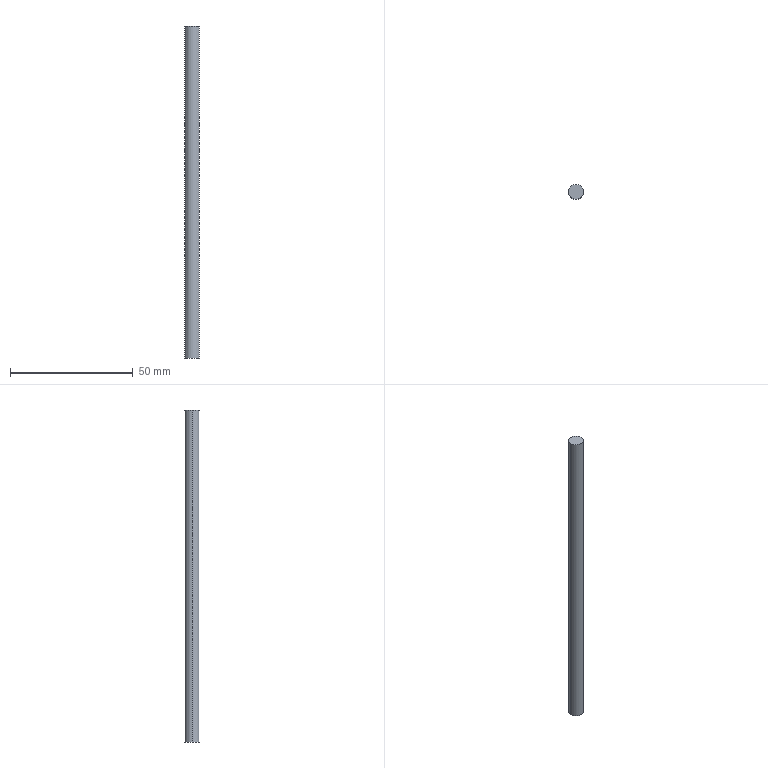Component | SolidWorks | Assembly5.1-1_TailstockAxisBar.1-1 | 1 solid | 4 faces | box 6 x 6 x 135 mm | volume 3817 mm3 | cylinder 2 | plane 2 | commonest cylinder face diameters 6 x2
build123d program:
from build123d import *

# Parameters (mm, degrees)
SKETCH1_R           = 3
BOSS_EXTRUDE1_DEPTH = 67.5


with BuildPart() as part:
    # Sketch1 → Boss-Extrude1 (new, symmetric)
    with BuildSketch(Plane.XY):
        Circle(SKETCH1_R)
    extrude(amount=BOSS_EXTRUDE1_DEPTH, both=True)


solid = part.part

# Placed as in the assembly
solid = solid.moved(Location((70, 164, 0), (0, 0, 0)))
STEP:
#1=COLOUR_RGB('',0.7922,0.8196,0.9333);
#2=FILL_AREA_STYLE_COLOUR('',#1);
#3=FILL_AREA_STYLE('',(#2));
#4=SURFACE_STYLE_FILL_AREA(#3);
#5=SURFACE_SIDE_STYLE('',(#4));
#6=SURFACE_STYLE_USAGE(.BOTH.,#5);
#7=PRESENTATION_STYLE_ASSIGNMENT((#6));
#8=CARTESIAN_POINT('',(2.874,6.457,2.657));
#9=VERTEX_POINT('',#8);
#10=CARTESIAN_POINT('',(2.638,6.457,2.657));
#11=VERTEX_POINT('',#10);
#12=CARTESIAN_POINT('',(2.756,6.457,2.657));
#13=DIRECTION('',(0.,0.,1.));
#14=DIRECTION('',(1.,0.,0.));
#15=AXIS2_PLACEMENT_3D('',#12,#13,#14);
#16=CIRCLE('',#15,0.1181);
#17=EDGE_CURVE('',#9,#11,#16,.T.);
#18=ORIENTED_EDGE('',*,*,#17,.F.);
#19=CARTESIAN_POINT('',(2.874,6.457,-2.657));
#20=VERTEX_POINT('',#19);
#21=CARTESIAN_POINT('',(2.874,6.457,2.657));
#22=DIRECTION('',(0.,0.,-1.));
#23=VECTOR('',#22,39.37);
#24=LINE('',#21,#23);
#25=EDGE_CURVE('',#9,#20,#24,.T.);
#26=ORIENTED_EDGE('',*,*,#25,.T.);
#27=CARTESIAN_POINT('',(2.638,6.457,-2.657));
#28=VERTEX_POINT('',#27);
#29=CARTESIAN_POINT('',(2.756,6.457,-2.657));
#30=DIRECTION('',(0.,0.,1.));
#31=DIRECTION('',(1.,0.,0.));
#32=AXIS2_PLACEMENT_3D('',#29,#30,#31);
#33=CIRCLE('',#32,0.1181);
#34=EDGE_CURVE('',#20,#28,#33,.T.);
#35=ORIENTED_EDGE('',*,*,#34,.T.);
#36=CARTESIAN_POINT('',(2.638,6.457,2.657));
#37=DIRECTION('',(0.,0.,-1.));
#38=VECTOR('',#37,39.37);
#39=LINE('',#36,#38);
#40=EDGE_CURVE('',#11,#28,#39,.T.);
#41=ORIENTED_EDGE('',*,*,#40,.F.);
#42=EDGE_LOOP('',(#18,#26,#35,#41));
#43=FACE_OUTER_BOUND('',#42,.T.);
#44=CARTESIAN_POINT('',(2.756,6.457,2.657));
#45=DIRECTION('',(0.,0.,-1.));
#46=DIRECTION('',(-1.,0.,0.));
#47=AXIS2_PLACEMENT_3D('',#44,#45,#46);
#48=CYLINDRICAL_SURFACE('',#47,0.1181);
#49=ADVANCED_FACE('',(#43),#48,.T.);
#50=ORIENTED_EDGE('',*,*,#25,.F.);
#51=CARTESIAN_POINT('',(2.756,6.457,2.657));
#52=DIRECTION('',(0.,0.,1.));
#53=DIRECTION('',(1.,0.,0.));
#54=AXIS2_PLACEMENT_3D('',#51,#52,#53);
#55=CIRCLE('',#54,0.1181);
#56=EDGE_CURVE('',#11,#9,#55,.T.);
#57=ORIENTED_EDGE('',*,*,#56,.F.);
#58=ORIENTED_EDGE('',*,*,#40,.T.);
#59=CARTESIAN_POINT('',(2.756,6.457,-2.657));
#60=DIRECTION('',(0.,0.,1.));
#61=DIRECTION('',(1.,0.,0.));
#62=AXIS2_PLACEMENT_3D('',#59,#60,#61);
#63=CIRCLE('',#62,0.1181);
#64=EDGE_CURVE('',#28,#20,#63,.T.);
#65=ORIENTED_EDGE('',*,*,#64,.T.);
#66=EDGE_LOOP('',(#50,#57,#58,#65));
#67=FACE_OUTER_BOUND('',#66,.T.);
#68=CARTESIAN_POINT('',(2.756,6.457,2.657));
#69=DIRECTION('',(0.,0.,-1.));
#70=DIRECTION('',(-1.,0.,0.));
#71=AXIS2_PLACEMENT_3D('',#68,#69,#70);
#72=CYLINDRICAL_SURFACE('',#71,0.1181);
#73=ADVANCED_FACE('',(#67),#72,.T.);
#74=ORIENTED_EDGE('',*,*,#56,.T.);
#75=ORIENTED_EDGE('',*,*,#17,.T.);
#76=EDGE_LOOP('',(#74,#75));
#77=FACE_OUTER_BOUND('',#76,.T.);
#78=CARTESIAN_POINT('',(2.756,6.457,2.657));
#79=DIRECTION('',(0.,0.,1.));
#80=DIRECTION('',(1.,0.,0.));
#81=AXIS2_PLACEMENT_3D('',#78,#79,#80);
#82=PLANE('',#81);
#83=ADVANCED_FACE('',(#77),#82,.T.);
#84=ORIENTED_EDGE('',*,*,#64,.F.);
#85=ORIENTED_EDGE('',*,*,#34,.F.);
#86=EDGE_LOOP('',(#84,#85));
#87=FACE_OUTER_BOUND('',#86,.T.);
#88=CARTESIAN_POINT('',(2.756,6.457,-2.657));
#89=DIRECTION('',(0.,0.,1.));
#90=DIRECTION('',(1.,0.,0.));
#91=AXIS2_PLACEMENT_3D('',#88,#89,#90);
#92=PLANE('',#91);
#93=ADVANCED_FACE('',(#87),#92,.F.);
#94=CLOSED_SHELL('',(#49,#73,#83,#93));
#95=MANIFOLD_SOLID_BREP('',#94);
#96=STYLED_ITEM('',(#7),#95);
#97=PRESENTATION_LAYER_ASSIGNMENT('','',(#96));
#98=(LENGTH_UNIT()NAMED_UNIT(*)SI_UNIT($,.METRE.));
#99=LENGTH_MEASURE_WITH_UNIT(LENGTH_MEASURE(0.0254),#98);
#100=DIMENSIONAL_EXPONENTS(1.,0.,0.,0.,0.,0.,0.);
#101=(CONVERSION_BASED_UNIT('',#99)LENGTH_UNIT()NAMED_UNIT(#100));
#102=UNCERTAINTY_MEASURE_WITH_UNIT(LENGTH_MEASURE(0.00001),#101,'','');
#103=(NAMED_UNIT(*)PLANE_ANGLE_UNIT()SI_UNIT($,.RADIAN.));
#104=(NAMED_UNIT(*)SI_UNIT($,.STERADIAN.)SOLID_ANGLE_UNIT());
#105=(GEOMETRIC_REPRESENTATION_CONTEXT(3)GLOBAL_UNCERTAINTY_ASSIGNED_CONTEXT((#102))GLOBAL_UNIT_ASSIGNED_CONTEXT((#101,#103,#104))REPRESENTATION_CONTEXT('',''));
#106=MECHANICAL_DESIGN_GEOMETRIC_PRESENTATION_REPRESENTATION('',(#96),#105);
#107=CARTESIAN_POINT('',(0.,0.,0.));
#108=DIRECTION('',(0.,0.,1.));
#109=DIRECTION('',(1.,0.,0.));
#110=AXIS2_PLACEMENT_3D('',#107,#108,#109);
#111=(LENGTH_UNIT()NAMED_UNIT(*)SI_UNIT($,.METRE.));
#112=LENGTH_MEASURE_WITH_UNIT(LENGTH_MEASURE(0.0254),#111);
#113=DIMENSIONAL_EXPONENTS(1.,0.,0.,0.,0.,0.,0.);
#114=(CONVERSION_BASED_UNIT('',#112)LENGTH_UNIT()NAMED_UNIT(#113));
#115=UNCERTAINTY_MEASURE_WITH_UNIT(LENGTH_MEASURE(0.00001),#114,'','');
#116=(NAMED_UNIT(*)PLANE_ANGLE_UNIT()SI_UNIT($,.RADIAN.));
#117=(NAMED_UNIT(*)SI_UNIT($,.STERADIAN.)SOLID_ANGLE_UNIT());
#118=(GEOMETRIC_REPRESENTATION_CONTEXT(3)GLOBAL_UNCERTAINTY_ASSIGNED_CONTEXT((#115))GLOBAL_UNIT_ASSIGNED_CONTEXT((#114,#116,#117))REPRESENTATION_CONTEXT('',''));
#119=ADVANCED_BREP_SHAPE_REPRESENTATION('',(#95,#110),#118);